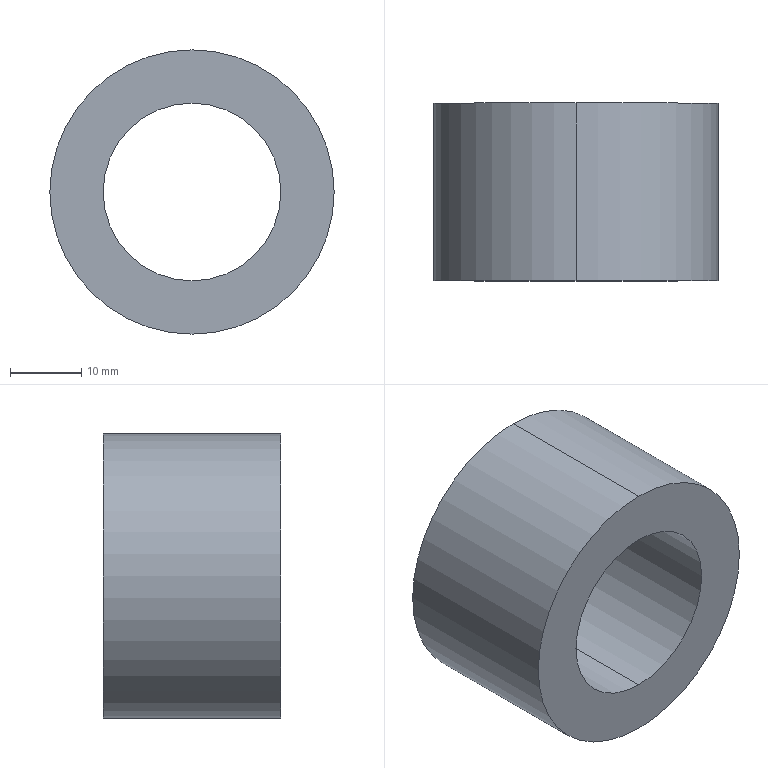Component | SolidWorks | THK-A1019FrontGuideWheelSpacerBlock-2 | 1 solid | 6 faces | box 40 x 25 x 40 mm | volume 19144 mm3 | cylinder 4 | plane 2 | commonest cylinder face diameters 25 x2 40 x2 | material Q235A
build123d program:
from build123d import *

# Parameters (mm, degrees)
SKETCH1_R           = 20
BOSS_EXTRUDE1_DEPTH = 12.5
SKETCH2_R           = 12.5
CUT_EXTRUDE1_DEPTH  = 38.749


with BuildPart() as part:
    # Sketch1 → Boss-Extrude1 (new, symmetric)
    with BuildSketch(Plane(origin=(0, 0, 0), x_dir=(1, 0, 0), z_dir=(0, 1, 0))):
        with Locations(Location((0, 0, 0), (0, 0, 270))):
            Circle(SKETCH1_R)
    extrude(amount=BOSS_EXTRUDE1_DEPTH, both=True)

    # Sketch2 → Cut-Extrude1 (cut, through all)
    with BuildSketch(Plane(origin=(0, 12.5, 0), x_dir=(1, 0, 0), z_dir=(0, 1, 0))):
        with Locations(Location((0, 0, 0), (0, 0, 270))):
            Circle(SKETCH2_R)
    extrude(amount=-CUT_EXTRUDE1_DEPTH, mode=Mode.SUBTRACT)


solid = part.part

# Placed as in the assembly
solid = solid.moved(Location((85, -116.5, -1181), (0, 0, 0)))
STEP:
#1=COLOUR_RGB('',0.7922,0.8196,0.9333);
#2=FILL_AREA_STYLE_COLOUR('',#1);
#3=FILL_AREA_STYLE('',(#2));
#4=SURFACE_STYLE_FILL_AREA(#3);
#5=SURFACE_SIDE_STYLE('',(#4));
#6=SURFACE_STYLE_USAGE(.BOTH.,#5);
#7=PRESENTATION_STYLE_ASSIGNMENT((#6));
#8=CARTESIAN_POINT('',(3.346,-5.079,-46.988));
#9=VERTEX_POINT('',#8);
#10=CARTESIAN_POINT('',(3.346,-5.079,-46.004));
#11=VERTEX_POINT('',#10);
#12=CARTESIAN_POINT('',(3.346,-5.079,-46.496));
#13=DIRECTION('',(0.,1.,-0.));
#14=DIRECTION('',(0.,0.,1.));
#15=AXIS2_PLACEMENT_3D('',#12,#13,#14);
#16=CIRCLE('',#15,0.4921);
#17=EDGE_CURVE('',#9,#11,#16,.T.);
#18=ORIENTED_EDGE('',*,*,#17,.F.);
#19=CARTESIAN_POINT('',(3.346,-4.094,-46.988));
#20=VERTEX_POINT('',#19);
#21=CARTESIAN_POINT('',(3.346,-5.079,-46.988));
#22=DIRECTION('',(0.,1.,-0.));
#23=VECTOR('',#22,39.37);
#24=LINE('',#21,#23);
#25=EDGE_CURVE('',#9,#20,#24,.T.);
#26=ORIENTED_EDGE('',*,*,#25,.T.);
#27=CARTESIAN_POINT('',(3.346,-4.094,-46.004));
#28=VERTEX_POINT('',#27);
#29=CARTESIAN_POINT('',(3.346,-4.094,-46.496));
#30=DIRECTION('',(0.,1.,-0.));
#31=DIRECTION('',(0.,0.,1.));
#32=AXIS2_PLACEMENT_3D('',#29,#30,#31);
#33=CIRCLE('',#32,0.4921);
#34=EDGE_CURVE('',#20,#28,#33,.T.);
#35=ORIENTED_EDGE('',*,*,#34,.T.);
#36=CARTESIAN_POINT('',(3.346,-5.079,-46.004));
#37=DIRECTION('',(0.,1.,-0.));
#38=VECTOR('',#37,39.37);
#39=LINE('',#36,#38);
#40=EDGE_CURVE('',#11,#28,#39,.T.);
#41=ORIENTED_EDGE('',*,*,#40,.F.);
#42=EDGE_LOOP('',(#18,#26,#35,#41));
#43=FACE_OUTER_BOUND('',#42,.T.);
#44=CARTESIAN_POINT('',(3.346,-5.079,-46.496));
#45=DIRECTION('',(0.,1.,-0.));
#46=DIRECTION('',(0.,0.,1.));
#47=AXIS2_PLACEMENT_3D('',#44,#45,#46);
#48=CYLINDRICAL_SURFACE('',#47,0.4921);
#49=ADVANCED_FACE('',(#43),#48,.F.);
#50=CARTESIAN_POINT('',(3.346,-4.094,-45.709));
#51=VERTEX_POINT('',#50);
#52=CARTESIAN_POINT('',(3.346,-4.094,-47.283));
#53=VERTEX_POINT('',#52);
#54=CARTESIAN_POINT('',(3.346,-4.094,-46.496));
#55=DIRECTION('',(0.,1.,-0.));
#56=DIRECTION('',(0.,0.,1.));
#57=AXIS2_PLACEMENT_3D('',#54,#55,#56);
#58=CIRCLE('',#57,0.7874);
#59=EDGE_CURVE('',#51,#53,#58,.T.);
#60=ORIENTED_EDGE('',*,*,#59,.F.);
#61=CARTESIAN_POINT('',(3.346,-5.079,-45.709));
#62=VERTEX_POINT('',#61);
#63=CARTESIAN_POINT('',(3.346,-4.094,-45.709));
#64=DIRECTION('',(0.,-1.,0.));
#65=VECTOR('',#64,39.37);
#66=LINE('',#63,#65);
#67=EDGE_CURVE('',#51,#62,#66,.T.);
#68=ORIENTED_EDGE('',*,*,#67,.T.);
#69=CARTESIAN_POINT('',(3.346,-5.079,-47.283));
#70=VERTEX_POINT('',#69);
#71=CARTESIAN_POINT('',(3.346,-5.079,-46.496));
#72=DIRECTION('',(0.,1.,-0.));
#73=DIRECTION('',(0.,0.,1.));
#74=AXIS2_PLACEMENT_3D('',#71,#72,#73);
#75=CIRCLE('',#74,0.7874);
#76=EDGE_CURVE('',#62,#70,#75,.T.);
#77=ORIENTED_EDGE('',*,*,#76,.T.);
#78=CARTESIAN_POINT('',(3.346,-4.094,-47.283));
#79=DIRECTION('',(0.,-1.,0.));
#80=VECTOR('',#79,39.37);
#81=LINE('',#78,#80);
#82=EDGE_CURVE('',#53,#70,#81,.T.);
#83=ORIENTED_EDGE('',*,*,#82,.F.);
#84=EDGE_LOOP('',(#60,#68,#77,#83));
#85=FACE_OUTER_BOUND('',#84,.T.);
#86=CARTESIAN_POINT('',(3.346,-4.094,-46.496));
#87=DIRECTION('',(0.,-1.,0.));
#88=DIRECTION('',(0.,0.,-1.));
#89=AXIS2_PLACEMENT_3D('',#86,#87,#88);
#90=CYLINDRICAL_SURFACE('',#89,0.7874);
#91=ADVANCED_FACE('',(#85),#90,.T.);
#92=ORIENTED_EDGE('',*,*,#67,.F.);
#93=CARTESIAN_POINT('',(3.346,-4.094,-46.496));
#94=DIRECTION('',(0.,1.,-0.));
#95=DIRECTION('',(0.,0.,1.));
#96=AXIS2_PLACEMENT_3D('',#93,#94,#95);
#97=CIRCLE('',#96,0.7874);
#98=EDGE_CURVE('',#53,#51,#97,.T.);
#99=ORIENTED_EDGE('',*,*,#98,.F.);
#100=ORIENTED_EDGE('',*,*,#82,.T.);
#101=CARTESIAN_POINT('',(3.346,-5.079,-46.496));
#102=DIRECTION('',(0.,1.,-0.));
#103=DIRECTION('',(0.,0.,1.));
#104=AXIS2_PLACEMENT_3D('',#101,#102,#103);
#105=CIRCLE('',#104,0.7874);
#106=EDGE_CURVE('',#70,#62,#105,.T.);
#107=ORIENTED_EDGE('',*,*,#106,.T.);
#108=EDGE_LOOP('',(#92,#99,#100,#107));
#109=FACE_OUTER_BOUND('',#108,.T.);
#110=CARTESIAN_POINT('',(3.346,-4.094,-46.496));
#111=DIRECTION('',(0.,-1.,0.));
#112=DIRECTION('',(0.,0.,-1.));
#113=AXIS2_PLACEMENT_3D('',#110,#111,#112);
#114=CYLINDRICAL_SURFACE('',#113,0.7874);
#115=ADVANCED_FACE('',(#109),#114,.T.);
#116=CARTESIAN_POINT('',(3.346,-4.094,-46.496));
#117=DIRECTION('',(0.,1.,-0.));
#118=DIRECTION('',(0.,0.,1.));
#119=AXIS2_PLACEMENT_3D('',#116,#117,#118);
#120=CIRCLE('',#119,0.4921);
#121=EDGE_CURVE('',#28,#20,#120,.T.);
#122=ORIENTED_EDGE('',*,*,#121,.F.);
#123=ORIENTED_EDGE('',*,*,#34,.F.);
#124=EDGE_LOOP('',(#122,#123));
#125=FACE_BOUND('',#124,.T.);
#126=ORIENTED_EDGE('',*,*,#98,.T.);
#127=ORIENTED_EDGE('',*,*,#59,.T.);
#128=EDGE_LOOP('',(#126,#127));
#129=FACE_OUTER_BOUND('',#128,.T.);
#130=CARTESIAN_POINT('',(3.346,-4.094,-46.496));
#131=DIRECTION('',(0.,1.,0.));
#132=DIRECTION('',(0.,-0.,1.));
#133=AXIS2_PLACEMENT_3D('',#130,#131,#132);
#134=PLANE('',#133);
#135=ADVANCED_FACE('',(#125,#129),#134,.T.);
#136=CARTESIAN_POINT('',(3.346,-5.079,-46.496));
#137=DIRECTION('',(0.,1.,-0.));
#138=DIRECTION('',(0.,0.,1.));
#139=AXIS2_PLACEMENT_3D('',#136,#137,#138);
#140=CIRCLE('',#139,0.4921);
#141=EDGE_CURVE('',#11,#9,#140,.T.);
#142=ORIENTED_EDGE('',*,*,#141,.T.);
#143=ORIENTED_EDGE('',*,*,#17,.T.);
#144=EDGE_LOOP('',(#142,#143));
#145=FACE_BOUND('',#144,.T.);
#146=ORIENTED_EDGE('',*,*,#106,.F.);
#147=ORIENTED_EDGE('',*,*,#76,.F.);
#148=EDGE_LOOP('',(#146,#147));
#149=FACE_OUTER_BOUND('',#148,.T.);
#150=CARTESIAN_POINT('',(3.346,-5.079,-46.496));
#151=DIRECTION('',(0.,1.,0.));
#152=DIRECTION('',(0.,-0.,1.));
#153=AXIS2_PLACEMENT_3D('',#150,#151,#152);
#154=PLANE('',#153);
#155=ADVANCED_FACE('',(#145,#149),#154,.F.);
#156=ORIENTED_EDGE('',*,*,#25,.F.);
#157=ORIENTED_EDGE('',*,*,#141,.F.);
#158=ORIENTED_EDGE('',*,*,#40,.T.);
#159=ORIENTED_EDGE('',*,*,#121,.T.);
#160=EDGE_LOOP('',(#156,#157,#158,#159));
#161=FACE_OUTER_BOUND('',#160,.T.);
#162=CARTESIAN_POINT('',(3.346,-5.079,-46.496));
#163=DIRECTION('',(0.,1.,-0.));
#164=DIRECTION('',(0.,0.,1.));
#165=AXIS2_PLACEMENT_3D('',#162,#163,#164);
#166=CYLINDRICAL_SURFACE('',#165,0.4921);
#167=ADVANCED_FACE('',(#161),#166,.F.);
#168=CLOSED_SHELL('',(#49,#91,#115,#135,#155,#167));
#169=MANIFOLD_SOLID_BREP('',#168);
#170=STYLED_ITEM('',(#7),#169);
#171=(LENGTH_UNIT()NAMED_UNIT(*)SI_UNIT($,.METRE.));
#172=LENGTH_MEASURE_WITH_UNIT(LENGTH_MEASURE(0.0254),#171);
#173=DIMENSIONAL_EXPONENTS(1.,0.,0.,0.,0.,0.,0.);
#174=(CONVERSION_BASED_UNIT('',#172)LENGTH_UNIT()NAMED_UNIT(#173));
#175=UNCERTAINTY_MEASURE_WITH_UNIT(LENGTH_MEASURE(0.00001),#174,'','');
#176=(NAMED_UNIT(*)PLANE_ANGLE_UNIT()SI_UNIT($,.RADIAN.));
#177=(NAMED_UNIT(*)SI_UNIT($,.STERADIAN.)SOLID_ANGLE_UNIT());
#178=(GEOMETRIC_REPRESENTATION_CONTEXT(3)GLOBAL_UNCERTAINTY_ASSIGNED_CONTEXT((#175))GLOBAL_UNIT_ASSIGNED_CONTEXT((#174,#176,#177))REPRESENTATION_CONTEXT('',''));
#179=MECHANICAL_DESIGN_GEOMETRIC_PRESENTATION_REPRESENTATION('',(#170),#178);
#180=PRESENTATION_LAYER_ASSIGNMENT('','',(#170));
#181=CARTESIAN_POINT('',(0.,0.,0.));
#182=DIRECTION('',(0.,0.,1.));
#183=DIRECTION('',(1.,0.,0.));
#184=AXIS2_PLACEMENT_3D('',#181,#182,#183);
#185=(LENGTH_UNIT()NAMED_UNIT(*)SI_UNIT($,.METRE.));
#186=LENGTH_MEASURE_WITH_UNIT(LENGTH_MEASURE(0.0254),#185);
#187=DIMENSIONAL_EXPONENTS(1.,0.,0.,0.,0.,0.,0.);
#188=(CONVERSION_BASED_UNIT('',#186)LENGTH_UNIT()NAMED_UNIT(#187));
#189=UNCERTAINTY_MEASURE_WITH_UNIT(LENGTH_MEASURE(0.00001),#188,'','');
#190=(NAMED_UNIT(*)PLANE_ANGLE_UNIT()SI_UNIT($,.RADIAN.));
#191=(NAMED_UNIT(*)SI_UNIT($,.STERADIAN.)SOLID_ANGLE_UNIT());
#192=(GEOMETRIC_REPRESENTATION_CONTEXT(3)GLOBAL_UNCERTAINTY_ASSIGNED_CONTEXT((#189))GLOBAL_UNIT_ASSIGNED_CONTEXT((#188,#190,#191))REPRESENTATION_CONTEXT('',''));
#193=ADVANCED_BREP_SHAPE_REPRESENTATION('',(#169,#184),#192);